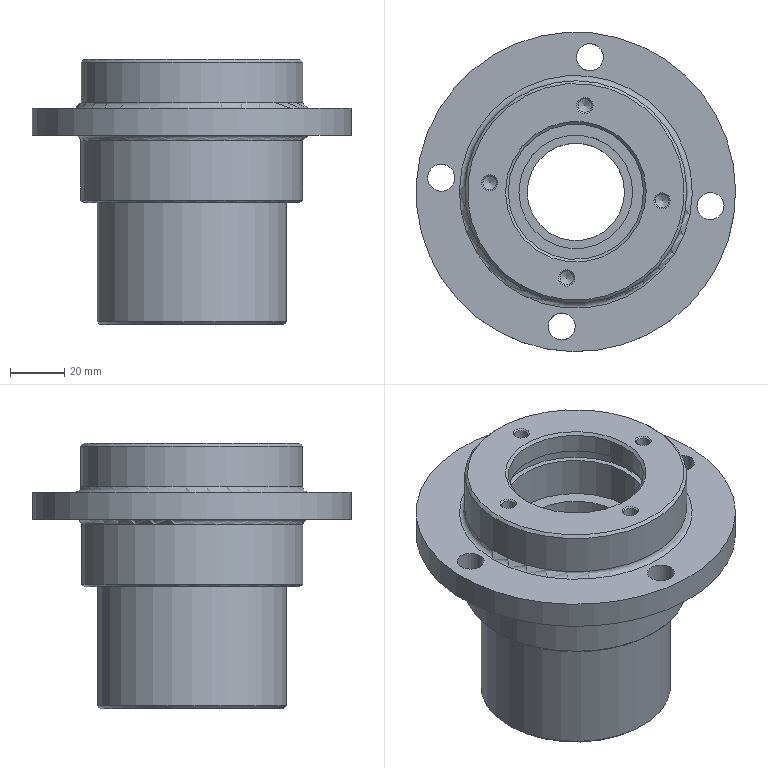Component | NX | FLANGE | 1 solid | 47 faces | volume 342360 mm3 | cylinder 20 | cone 13 | plane 12 | torus 2 | commonest cylinder face diameters 5 x4 10 x4 82 x2 52 x2 50 x2 118 x1 36 x1 54 x1